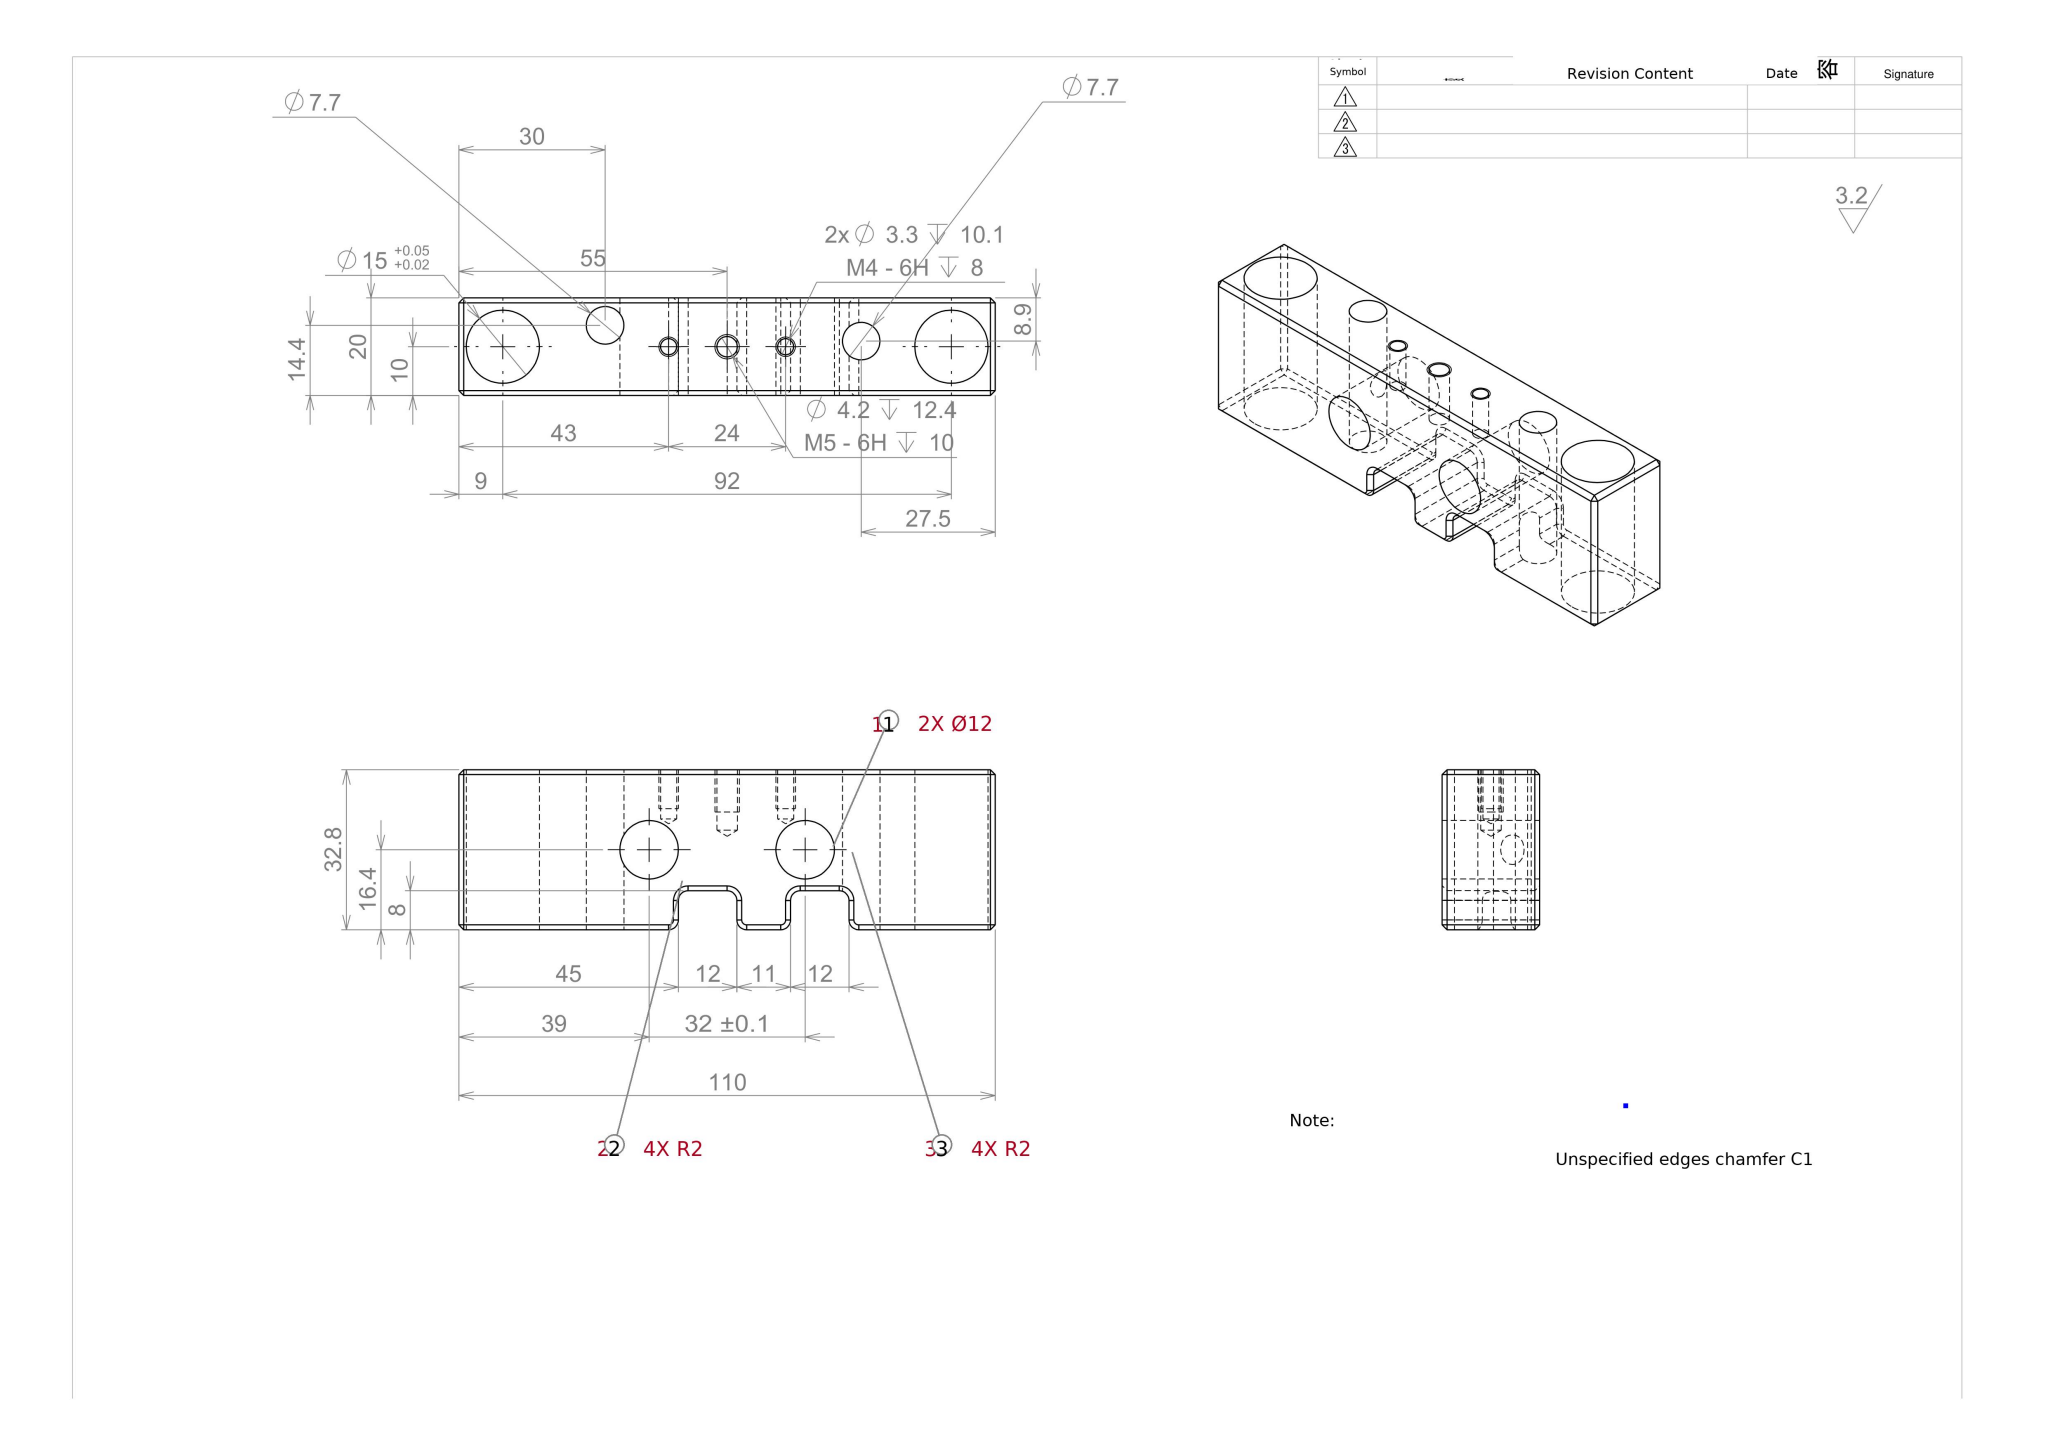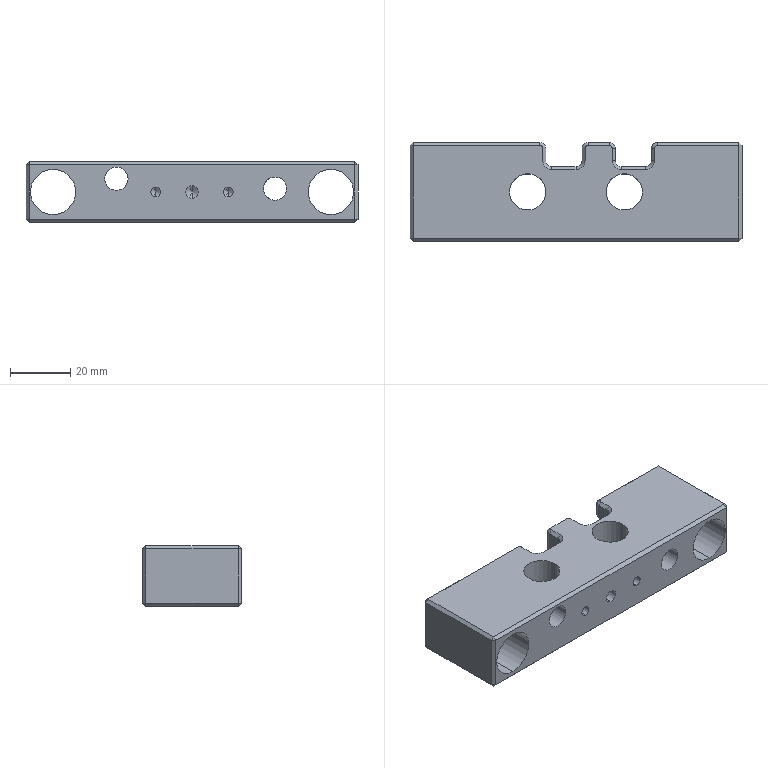Part | SolidWorks | mm | 1 solid | 100 faces | box 110 x 32.8 x 20 mm | volume 48499 mm3 | plane 51 | cylinder 27 | cone 22 | commonest cylinder face diameters 4 x9 12 x4 3.3 x4 15 x4 7.717 x2 7.691 x2 4.2 x2
build123d program:
from build123d import *

# Parameters (mm, degrees)
SKETCH1_W             = 110
SKETCH1_H             = 32.8
BOSS_EXTRUDE1_DEPTH   = 20
SKETCH4_R             = 7.5
CUT_EXTRUDE2_DEPTH    = 68.088
M5_TAPPED_HOLE1_D     = 4.2
M5_TAPPED_HOLE1_DEPTH = 12.4
M5_TAPPED_HOLE1_TIP   = 1.262
M4_TAPPED_HOLE1_D     = 3.3
M4_TAPPED_HOLE1_DEPTH = 10.1
M4_TAPPED_HOLE1_TIP   = 0.9914
M4_TAPPED_HOLE2_D     = 3.3
M4_TAPPED_HOLE2_DEPTH = 10.1
M4_TAPPED_HOLE2_TIP   = 0.9914
SKETCH9_R             = 6
CUT_EXTRUDE3_DEPTH    = 61.778
SKETCH10_W            = 12
SKETCH10_H            = 8
CUT_EXTRUDE4_DEPTH    = 61.778
FILLET1_R             = 2
CHAMFER1_SIZE         = 1
SKETCH11_R            = 3.859
SKETCH11_R_2          = 3.846
CUT_EXTRUDE5_DEPTH    = 40


with BuildPart() as part:
    # Sketch1 → Boss-Extrude1 (new body)
    with BuildSketch(Plane.XY):
        Rectangle(SKETCH1_W, SKETCH1_H)
    extrude(amount=BOSS_EXTRUDE1_DEPTH)

    # Sketch4 → Cut-Extrude2 (cut, through all)
    with BuildSketch(Plane.XZ.offset(16.4)):
        with Locations(Location((-46, 10, 0), (0, 0, 270))):
            Circle(SKETCH4_R)
        with Locations(Location((46, 10, 0), (0, 0, 270))):
            Circle(SKETCH4_R)
    extrude(amount=-CUT_EXTRUDE2_DEPTH, mode=Mode.SUBTRACT)

    # M5 Tapped Hole1
    with Locations(Plane(origin=(0, -16.4, 10), x_dir=(-1, 0, 0), z_dir=(0, -1, 0))):
        with Locations((0, 0)):
            Hole(M5_TAPPED_HOLE1_D / 2, depth=M5_TAPPED_HOLE1_DEPTH)
            with Locations((0, 0, -(M5_TAPPED_HOLE1_DEPTH + M5_TAPPED_HOLE1_TIP / 2))):  # 118° drill point
                Cone(0, M5_TAPPED_HOLE1_D / 2, M5_TAPPED_HOLE1_TIP, mode=Mode.SUBTRACT)

    # M4 Tapped Hole1
    with Locations(Plane(origin=(20, 0, 0), x_dir=(-1, 0, 0), z_dir=(0, 0, -1))):
        with Locations((0, 0)):
            Hole(M4_TAPPED_HOLE1_D / 2, depth=M4_TAPPED_HOLE1_DEPTH)
            with Locations((0, 0, -(M4_TAPPED_HOLE1_DEPTH + M4_TAPPED_HOLE1_TIP / 2))):  # 118° drill point
                Cone(0, M4_TAPPED_HOLE1_D / 2, M4_TAPPED_HOLE1_TIP, mode=Mode.SUBTRACT)

    # M4 Tapped Hole2
    with Locations(Plane(origin=(-12, -16.4, 10), x_dir=(-1, 0, 0), z_dir=(0, -1, 0))):
        with Locations((0, 0), (-24, 0)):
            Hole(M4_TAPPED_HOLE2_D / 2, depth=M4_TAPPED_HOLE2_DEPTH)
            with Locations((0, 0, -(M4_TAPPED_HOLE2_DEPTH + M4_TAPPED_HOLE2_TIP / 2))):  # 118° drill point
                Cone(0, M4_TAPPED_HOLE2_D / 2, M4_TAPPED_HOLE2_TIP, mode=Mode.SUBTRACT)

    # Sketch9 → Cut-Extrude3 (cut, through all)
    with BuildSketch(Plane.XY.offset(20)):
        with Locations((16, 0)):
            Circle(SKETCH9_R)
        with Locations(Location((-16, 0, 0), (0, 0, 180))):
            Circle(SKETCH9_R)
    extrude(amount=-CUT_EXTRUDE3_DEPTH, mode=Mode.SUBTRACT)

    # Sketch10 → Cut-Extrude4 (cut, through all)
    with BuildSketch(Plane.XY.offset(20)):
        with Locations((19, 12.4)):
            Rectangle(SKETCH10_W, SKETCH10_H)
        with Locations((-4, 12.4)):
            Rectangle(SKETCH10_W, SKETCH10_H)
    extrude(amount=-CUT_EXTRUDE4_DEPTH, mode=Mode.SUBTRACT)

    # Fillet1
    fillet1_edges = [part.edges().sort_by_distance(p)[0] for p in [
        (13, 8.4, 10),
        (13, 16.4, 10),
        (25, 16.4, 10),
        (25, 8.4, 10),
        (-10, 8.4, 10),
        (-10, 16.4, 10),
        (2, 16.4, 10),
        (2, 8.4, 10),
    ]]
    fillet(fillet1_edges, radius=FILLET1_R)

    # Chamfer1
    chamfer1_edges = [part.edges().sort_by_distance(p)[0] for p in [
        (0, -16.4, 20),
        (-9.414, 8.986, 20),
        (-9.414, 8.986, 0),
        (1.414, 8.986, 20),
        (1.414, 8.986, 0),
        (13.586, 8.986, 20),
        (13.586, 8.986, 0),
        (24.414, 8.986, 20),
        (24.414, 8.986, 0),
        (55, 0, 20),
        (41, 16.4, 20),
        (55, 0, 0),
        (0, -16.4, 0),
        (-55, 0, 0),
        (41, 16.4, 0),
        (-55, 0, 20),
        (55, 16.4, 10),
        (55, -16.4, 10),
        (-55, -16.4, 10),
        (-55, 16.4, 10),
        (-10, 12.4, 20),
        (-10, 12.4, 0),
        (-4, 8.4, 20),
        (-33.5, 16.4, 20),
        (25, 12.4, 20),
        (19, 8.4, 20),
        (13, 12.4, 20),
        (7.5, 16.4, 20),
        (2, 12.4, 20),
        (25.586, 15.814, 20),
        (12.414, 15.814, 20),
        (2.586, 15.814, 20),
        (-10.586, 15.814, 20),
        (-33.5, 16.4, 0),
        (-4, 8.4, 0),
        (2, 12.4, 0),
        (7.5, 16.4, 0),
        (13, 12.4, 0),
        (19, 8.4, 0),
        (25, 12.4, 0),
        (25.586, 15.814, 0),
        (12.414, 15.814, 0),
        (2.586, 15.814, 0),
        (-10.586, 15.814, 0),
    ]]
    chamfer(chamfer1_edges, length=CHAMFER1_SIZE)

    # Sketch11 → Cut-Extrude5 (cut)
    with BuildSketch(Plane.XZ.offset(16.4)):
        with Locations((-25.027, 14.384)):
            Circle(SKETCH11_R)
        with Locations((27.5, 11.146)):
            Circle(SKETCH11_R_2)
    extrude(amount=-CUT_EXTRUDE5_DEPTH, mode=Mode.SUBTRACT)


solid = part.part